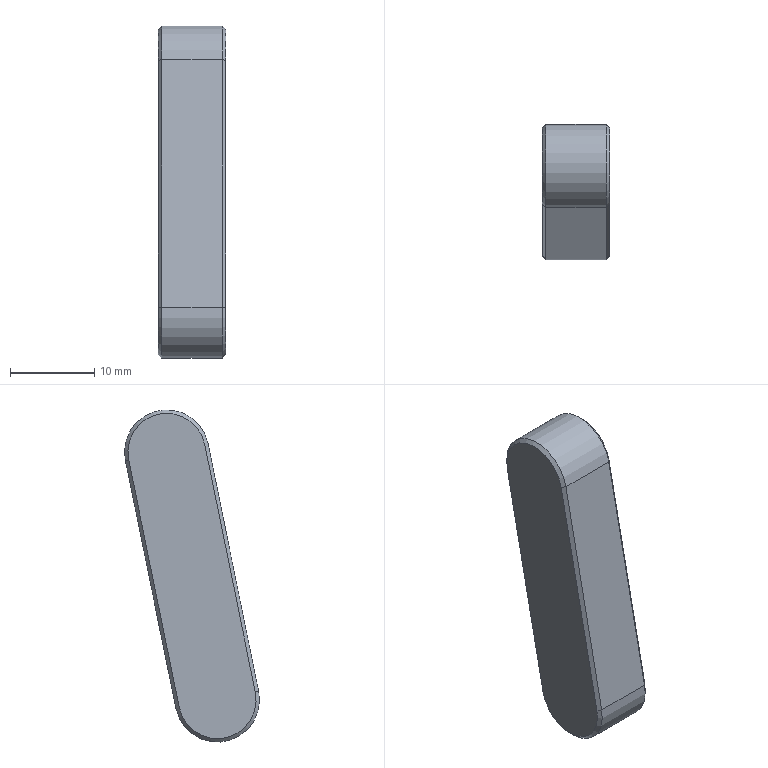Component | SolidWorks | Key_10-40-1 | 1 solid | 14 faces | box 8 x 16 x 39.39 mm | volume 3014 mm3 | plane 8 | cone 4 | cylinder 2 | commonest cylinder face diameters 10 x2
STEP:
#1=COLOUR_RGB('',0.7922,0.8196,0.9333);
#2=FILL_AREA_STYLE_COLOUR('',#1);
#3=FILL_AREA_STYLE('',(#2));
#4=SURFACE_STYLE_FILL_AREA(#3);
#5=SURFACE_SIDE_STYLE('',(#4));
#6=SURFACE_STYLE_USAGE(.BOTH.,#5);
#7=PRESENTATION_STYLE_ASSIGNMENT((#6));
#8=CARTESIAN_POINT('',(0.6063,7.591,5.523));
#9=VERTEX_POINT('',#8);
#10=CARTESIAN_POINT('',(0.8898,7.591,5.523));
#11=VERTEX_POINT('',#10);
#12=CARTESIAN_POINT('',(0.5906,7.591,5.523));
#13=DIRECTION('',(1.,-0.,-0.));
#14=VECTOR('',#13,39.37);
#15=LINE('',#12,#14);
#16=EDGE_CURVE('',#9,#11,#15,.T.);
#17=ORIENTED_EDGE('',*,*,#16,.T.);
#18=CARTESIAN_POINT('',(0.8898,7.828,6.68));
#19=VERTEX_POINT('',#18);
#20=CARTESIAN_POINT('',(0.8898,7.828,6.68));
#21=DIRECTION('',(0.,0.2,0.9798));
#22=VECTOR('',#21,39.37);
#23=LINE('',#20,#22);
#24=EDGE_CURVE('',#11,#19,#23,.T.);
#25=ORIENTED_EDGE('',*,*,#24,.T.);
#26=CARTESIAN_POINT('',(0.6063,7.828,6.68));
#27=VERTEX_POINT('',#26);
#28=CARTESIAN_POINT('',(0.5906,7.828,6.68));
#29=DIRECTION('',(1.,-0.,-0.));
#30=VECTOR('',#29,39.37);
#31=LINE('',#28,#30);
#32=EDGE_CURVE('',#27,#19,#31,.T.);
#33=ORIENTED_EDGE('',*,*,#32,.F.);
#34=CARTESIAN_POINT('',(0.6063,7.552,5.33));
#35=DIRECTION('',(-0.,-0.2,-0.9798));
#36=VECTOR('',#35,39.37);
#37=LINE('',#34,#36);
#38=EDGE_CURVE('',#27,#9,#37,.T.);
#39=ORIENTED_EDGE('',*,*,#38,.T.);
#40=EDGE_LOOP('',(#17,#25,#33,#39));
#41=FACE_OUTER_BOUND('',#40,.T.);
#42=CARTESIAN_POINT('',(0.5906,7.552,5.33));
#43=DIRECTION('',(-0.,0.9798,-0.2));
#44=DIRECTION('',(-0.,-0.2,-0.9798));
#45=AXIS2_PLACEMENT_3D('',#42,#43,#44);
#46=PLANE('',#45);
#47=ADVANCED_FACE('',(#41),#46,.F.);
#48=CARTESIAN_POINT('',(0.6063,8.213,6.601));
#49=VERTEX_POINT('',#48);
#50=CARTESIAN_POINT('',(0.8898,8.213,6.601));
#51=VERTEX_POINT('',#50);
#52=CARTESIAN_POINT('',(0.5906,8.213,6.601));
#53=DIRECTION('',(1.,-0.,-0.));
#54=VECTOR('',#53,39.37);
#55=LINE('',#52,#54);
#56=EDGE_CURVE('',#49,#51,#55,.T.);
#57=ORIENTED_EDGE('',*,*,#56,.T.);
#58=CARTESIAN_POINT('',(0.8898,7.977,5.444));
#59=VERTEX_POINT('',#58);
#60=CARTESIAN_POINT('',(0.8898,7.977,5.444));
#61=DIRECTION('',(-0.,-0.2,-0.9798));
#62=VECTOR('',#61,39.37);
#63=LINE('',#60,#62);
#64=EDGE_CURVE('',#51,#59,#63,.T.);
#65=ORIENTED_EDGE('',*,*,#64,.T.);
#66=CARTESIAN_POINT('',(0.6063,7.977,5.444));
#67=VERTEX_POINT('',#66);
#68=CARTESIAN_POINT('',(0.5906,7.977,5.444));
#69=DIRECTION('',(1.,-0.,-0.));
#70=VECTOR('',#69,39.37);
#71=LINE('',#68,#70);
#72=EDGE_CURVE('',#67,#59,#71,.T.);
#73=ORIENTED_EDGE('',*,*,#72,.F.);
#74=CARTESIAN_POINT('',(0.6063,7.938,5.251));
#75=DIRECTION('',(0.,0.2,0.9798));
#76=VECTOR('',#75,39.37);
#77=LINE('',#74,#76);
#78=EDGE_CURVE('',#67,#49,#77,.T.);
#79=ORIENTED_EDGE('',*,*,#78,.T.);
#80=EDGE_LOOP('',(#57,#65,#73,#79));
#81=FACE_OUTER_BOUND('',#80,.T.);
#82=CARTESIAN_POINT('',(0.5906,7.938,5.251));
#83=DIRECTION('',(0.,-0.9798,0.2));
#84=DIRECTION('',(0.,0.2,0.9798));
#85=AXIS2_PLACEMENT_3D('',#82,#83,#84);
#86=PLANE('',#85);
#87=ADVANCED_FACE('',(#81),#86,.F.);
#88=CARTESIAN_POINT('',(0.5906,7.843,6.677));
#89=VERTEX_POINT('',#88);
#90=CARTESIAN_POINT('',(0.5906,8.198,6.604));
#91=VERTEX_POINT('',#90);
#92=CARTESIAN_POINT('',(0.5906,8.02,6.64));
#93=DIRECTION('',(-1.,0.,0.));
#94=DIRECTION('',(0.,0.9798,-0.2));
#95=AXIS2_PLACEMENT_3D('',#92,#93,#94);
#96=CIRCLE('',#95,0.1811);
#97=EDGE_CURVE('',#89,#91,#96,.T.);
#98=ORIENTED_EDGE('',*,*,#97,.T.);
#99=CARTESIAN_POINT('',(0.5906,7.962,5.447));
#100=VERTEX_POINT('',#99);
#101=CARTESIAN_POINT('',(0.5906,7.922,5.254));
#102=DIRECTION('',(-0.,-0.2,-0.9798));
#103=VECTOR('',#102,39.37);
#104=LINE('',#101,#103);
#105=EDGE_CURVE('',#91,#100,#104,.T.);
#106=ORIENTED_EDGE('',*,*,#105,.T.);
#107=CARTESIAN_POINT('',(0.5906,7.607,5.519));
#108=VERTEX_POINT('',#107);
#109=CARTESIAN_POINT('',(0.5906,7.784,5.483));
#110=DIRECTION('',(-1.,0.,0.));
#111=DIRECTION('',(0.,0.9798,-0.2));
#112=AXIS2_PLACEMENT_3D('',#109,#110,#111);
#113=CIRCLE('',#112,0.1811);
#114=EDGE_CURVE('',#100,#108,#113,.T.);
#115=ORIENTED_EDGE('',*,*,#114,.T.);
#116=CARTESIAN_POINT('',(0.5906,7.568,5.326));
#117=DIRECTION('',(0.,0.2,0.9798));
#118=VECTOR('',#117,39.37);
#119=LINE('',#116,#118);
#120=EDGE_CURVE('',#108,#89,#119,.T.);
#121=ORIENTED_EDGE('',*,*,#120,.T.);
#122=EDGE_LOOP('',(#98,#106,#115,#121));
#123=FACE_OUTER_BOUND('',#122,.T.);
#124=CARTESIAN_POINT('',(0.5906,7.938,5.251));
#125=DIRECTION('',(1.,-0.,-0.));
#126=DIRECTION('',(0.,0.9798,-0.2));
#127=AXIS2_PLACEMENT_3D('',#124,#125,#126);
#128=PLANE('',#127);
#129=ADVANCED_FACE('',(#123),#128,.F.);
#130=CARTESIAN_POINT('',(0.9055,7.843,6.677));
#131=VERTEX_POINT('',#130);
#132=CARTESIAN_POINT('',(0.9055,7.607,5.519));
#133=VERTEX_POINT('',#132);
#134=CARTESIAN_POINT('',(0.9055,7.607,5.519));
#135=DIRECTION('',(-0.,-0.2,-0.9798));
#136=VECTOR('',#135,39.37);
#137=LINE('',#134,#136);
#138=EDGE_CURVE('',#131,#133,#137,.T.);
#139=ORIENTED_EDGE('',*,*,#138,.T.);
#140=CARTESIAN_POINT('',(0.9055,7.962,5.447));
#141=VERTEX_POINT('',#140);
#142=CARTESIAN_POINT('',(0.9055,7.784,5.483));
#143=DIRECTION('',(1.,-0.,-0.));
#144=DIRECTION('',(0.,0.9798,-0.2));
#145=AXIS2_PLACEMENT_3D('',#142,#143,#144);
#146=CIRCLE('',#145,0.1811);
#147=EDGE_CURVE('',#133,#141,#146,.T.);
#148=ORIENTED_EDGE('',*,*,#147,.T.);
#149=CARTESIAN_POINT('',(0.9055,8.198,6.604));
#150=VERTEX_POINT('',#149);
#151=CARTESIAN_POINT('',(0.9055,8.198,6.604));
#152=DIRECTION('',(0.,0.2,0.9798));
#153=VECTOR('',#152,39.37);
#154=LINE('',#151,#153);
#155=EDGE_CURVE('',#141,#150,#154,.T.);
#156=ORIENTED_EDGE('',*,*,#155,.T.);
#157=CARTESIAN_POINT('',(0.9055,8.02,6.64));
#158=DIRECTION('',(1.,-0.,-0.));
#159=DIRECTION('',(0.,0.9798,-0.2));
#160=AXIS2_PLACEMENT_3D('',#157,#158,#159);
#161=CIRCLE('',#160,0.1811);
#162=EDGE_CURVE('',#150,#131,#161,.T.);
#163=ORIENTED_EDGE('',*,*,#162,.T.);
#164=EDGE_LOOP('',(#139,#148,#156,#163));
#165=FACE_OUTER_BOUND('',#164,.T.);
#166=CARTESIAN_POINT('',(0.9055,7.938,5.251));
#167=DIRECTION('',(1.,-0.,-0.));
#168=DIRECTION('',(0.,0.9798,-0.2));
#169=AXIS2_PLACEMENT_3D('',#166,#167,#168);
#170=PLANE('',#169);
#171=ADVANCED_FACE('',(#165),#170,.T.);
#172=ORIENTED_EDGE('',*,*,#32,.T.);
#173=CARTESIAN_POINT('',(0.8898,8.02,6.64));
#174=DIRECTION('',(-1.,0.,0.));
#175=DIRECTION('',(0.,0.9798,-0.2));
#176=AXIS2_PLACEMENT_3D('',#173,#174,#175);
#177=CIRCLE('',#176,0.1969);
#178=EDGE_CURVE('',#19,#51,#177,.T.);
#179=ORIENTED_EDGE('',*,*,#178,.T.);
#180=ORIENTED_EDGE('',*,*,#56,.F.);
#181=CARTESIAN_POINT('',(0.6063,8.02,6.64));
#182=DIRECTION('',(1.,-0.,-0.));
#183=DIRECTION('',(0.,0.9798,-0.2));
#184=AXIS2_PLACEMENT_3D('',#181,#182,#183);
#185=CIRCLE('',#184,0.1969);
#186=EDGE_CURVE('',#49,#27,#185,.T.);
#187=ORIENTED_EDGE('',*,*,#186,.T.);
#188=EDGE_LOOP('',(#172,#179,#180,#187));
#189=FACE_OUTER_BOUND('',#188,.T.);
#190=CARTESIAN_POINT('',(0.5906,8.02,6.64));
#191=DIRECTION('',(1.,-0.,-0.));
#192=DIRECTION('',(0.,0.9798,-0.2));
#193=AXIS2_PLACEMENT_3D('',#190,#191,#192);
#194=CYLINDRICAL_SURFACE('',#193,0.1969);
#195=ADVANCED_FACE('',(#189),#194,.T.);
#196=ORIENTED_EDGE('',*,*,#72,.T.);
#197=CARTESIAN_POINT('',(0.8898,7.784,5.483));
#198=DIRECTION('',(-1.,0.,0.));
#199=DIRECTION('',(0.,0.9798,-0.2));
#200=AXIS2_PLACEMENT_3D('',#197,#198,#199);
#201=CIRCLE('',#200,0.1969);
#202=EDGE_CURVE('',#59,#11,#201,.T.);
#203=ORIENTED_EDGE('',*,*,#202,.T.);
#204=ORIENTED_EDGE('',*,*,#16,.F.);
#205=CARTESIAN_POINT('',(0.6063,7.784,5.483));
#206=DIRECTION('',(1.,-0.,-0.));
#207=DIRECTION('',(0.,0.9798,-0.2));
#208=AXIS2_PLACEMENT_3D('',#205,#206,#207);
#209=CIRCLE('',#208,0.1969);
#210=EDGE_CURVE('',#9,#67,#209,.T.);
#211=ORIENTED_EDGE('',*,*,#210,.T.);
#212=EDGE_LOOP('',(#196,#203,#204,#211));
#213=FACE_OUTER_BOUND('',#212,.T.);
#214=CARTESIAN_POINT('',(0.5906,7.784,5.483));
#215=DIRECTION('',(1.,-0.,-0.));
#216=DIRECTION('',(0.,0.9798,-0.2));
#217=AXIS2_PLACEMENT_3D('',#214,#215,#216);
#218=CYLINDRICAL_SURFACE('',#217,0.1969);
#219=ADVANCED_FACE('',(#213),#218,.T.);
#220=CARTESIAN_POINT('',(0.9055,7.843,6.677));
#221=DIRECTION('',(-0.7071,-0.6928,0.1414));
#222=VECTOR('',#221,39.37);
#223=LINE('',#220,#222);
#224=EDGE_CURVE('',#131,#19,#223,.T.);
#225=ORIENTED_EDGE('',*,*,#224,.F.);
#226=ORIENTED_EDGE('',*,*,#162,.F.);
#227=CARTESIAN_POINT('',(0.8898,8.213,6.601));
#228=DIRECTION('',(0.7071,-0.6928,0.1414));
#229=VECTOR('',#228,39.37);
#230=LINE('',#227,#229);
#231=EDGE_CURVE('',#51,#150,#230,.T.);
#232=ORIENTED_EDGE('',*,*,#231,.F.);
#233=ORIENTED_EDGE('',*,*,#178,.F.);
#234=EDGE_LOOP('',(#225,#226,#232,#233));
#235=FACE_OUTER_BOUND('',#234,.T.);
#236=CARTESIAN_POINT('',(0.8898,8.02,6.64));
#237=DIRECTION('',(-1.,0.,0.));
#238=DIRECTION('',(0.,-0.9798,0.2));
#239=AXIS2_PLACEMENT_3D('',#236,#237,#238);
#240=CONICAL_SURFACE('',#239,0.1969,0.7854);
#241=ADVANCED_FACE('',(#235),#240,.T.);
#242=ORIENTED_EDGE('',*,*,#231,.T.);
#243=ORIENTED_EDGE('',*,*,#155,.F.);
#244=CARTESIAN_POINT('',(0.8898,7.977,5.444));
#245=DIRECTION('',(0.7071,-0.6928,0.1414));
#246=VECTOR('',#245,39.37);
#247=LINE('',#244,#246);
#248=EDGE_CURVE('',#59,#141,#247,.T.);
#249=ORIENTED_EDGE('',*,*,#248,.F.);
#250=ORIENTED_EDGE('',*,*,#64,.F.);
#251=EDGE_LOOP('',(#242,#243,#249,#250));
#252=FACE_OUTER_BOUND('',#251,.T.);
#253=CARTESIAN_POINT('',(0.8898,7.938,5.251));
#254=DIRECTION('',(0.7071,0.6928,-0.1414));
#255=DIRECTION('',(-0.7071,0.6928,-0.1414));
#256=AXIS2_PLACEMENT_3D('',#253,#254,#255);
#257=PLANE('',#256);
#258=ADVANCED_FACE('',(#252),#257,.T.);
#259=ORIENTED_EDGE('',*,*,#224,.T.);
#260=ORIENTED_EDGE('',*,*,#24,.F.);
#261=CARTESIAN_POINT('',(0.9055,7.607,5.519));
#262=DIRECTION('',(-0.7071,-0.6928,0.1414));
#263=VECTOR('',#262,39.37);
#264=LINE('',#261,#263);
#265=EDGE_CURVE('',#133,#11,#264,.T.);
#266=ORIENTED_EDGE('',*,*,#265,.F.);
#267=ORIENTED_EDGE('',*,*,#138,.F.);
#268=EDGE_LOOP('',(#259,#260,#266,#267));
#269=FACE_OUTER_BOUND('',#268,.T.);
#270=CARTESIAN_POINT('',(0.8898,7.552,5.33));
#271=DIRECTION('',(0.7071,-0.6928,0.1414));
#272=DIRECTION('',(0.7071,0.6928,-0.1414));
#273=AXIS2_PLACEMENT_3D('',#270,#271,#272);
#274=PLANE('',#273);
#275=ADVANCED_FACE('',(#269),#274,.T.);
#276=ORIENTED_EDGE('',*,*,#248,.T.);
#277=ORIENTED_EDGE('',*,*,#147,.F.);
#278=ORIENTED_EDGE('',*,*,#265,.T.);
#279=ORIENTED_EDGE('',*,*,#202,.F.);
#280=EDGE_LOOP('',(#276,#277,#278,#279));
#281=FACE_OUTER_BOUND('',#280,.T.);
#282=CARTESIAN_POINT('',(0.8898,7.784,5.483));
#283=DIRECTION('',(-1.,0.,0.));
#284=DIRECTION('',(0.,-0.9798,0.2));
#285=AXIS2_PLACEMENT_3D('',#282,#283,#284);
#286=CONICAL_SURFACE('',#285,0.1969,0.7854);
#287=ADVANCED_FACE('',(#281),#286,.T.);
#288=CARTESIAN_POINT('',(0.6063,7.591,5.523));
#289=DIRECTION('',(-0.7071,0.6928,-0.1414));
#290=VECTOR('',#289,39.37);
#291=LINE('',#288,#290);
#292=EDGE_CURVE('',#9,#108,#291,.T.);
#293=ORIENTED_EDGE('',*,*,#292,.F.);
#294=ORIENTED_EDGE('',*,*,#38,.F.);
#295=CARTESIAN_POINT('',(0.5906,7.843,6.677));
#296=DIRECTION('',(0.7071,-0.6928,0.1414));
#297=VECTOR('',#296,39.37);
#298=LINE('',#295,#297);
#299=EDGE_CURVE('',#89,#27,#298,.T.);
#300=ORIENTED_EDGE('',*,*,#299,.F.);
#301=ORIENTED_EDGE('',*,*,#120,.F.);
#302=EDGE_LOOP('',(#293,#294,#300,#301));
#303=FACE_OUTER_BOUND('',#302,.T.);
#304=CARTESIAN_POINT('',(0.5906,7.568,5.326));
#305=DIRECTION('',(0.7071,0.6928,-0.1414));
#306=DIRECTION('',(-0.7071,0.6928,-0.1414));
#307=AXIS2_PLACEMENT_3D('',#304,#305,#306);
#308=PLANE('',#307);
#309=ADVANCED_FACE('',(#303),#308,.F.);
#310=ORIENTED_EDGE('',*,*,#299,.T.);
#311=ORIENTED_EDGE('',*,*,#186,.F.);
#312=CARTESIAN_POINT('',(0.5906,8.198,6.604));
#313=DIRECTION('',(0.7071,0.6928,-0.1414));
#314=VECTOR('',#313,39.37);
#315=LINE('',#312,#314);
#316=EDGE_CURVE('',#91,#49,#315,.T.);
#317=ORIENTED_EDGE('',*,*,#316,.F.);
#318=ORIENTED_EDGE('',*,*,#97,.F.);
#319=EDGE_LOOP('',(#310,#311,#317,#318));
#320=FACE_OUTER_BOUND('',#319,.T.);
#321=CARTESIAN_POINT('',(0.5906,8.02,6.64));
#322=DIRECTION('',(1.,-0.,-0.));
#323=DIRECTION('',(0.,0.9798,-0.2));
#324=AXIS2_PLACEMENT_3D('',#321,#322,#323);
#325=CONICAL_SURFACE('',#324,0.1811,0.7854);
#326=ADVANCED_FACE('',(#320),#325,.T.);
#327=ORIENTED_EDGE('',*,*,#292,.T.);
#328=ORIENTED_EDGE('',*,*,#114,.F.);
#329=CARTESIAN_POINT('',(0.6063,7.977,5.444));
#330=DIRECTION('',(-0.7071,-0.6928,0.1414));
#331=VECTOR('',#330,39.37);
#332=LINE('',#329,#331);
#333=EDGE_CURVE('',#67,#100,#332,.T.);
#334=ORIENTED_EDGE('',*,*,#333,.F.);
#335=ORIENTED_EDGE('',*,*,#210,.F.);
#336=EDGE_LOOP('',(#327,#328,#334,#335));
#337=FACE_OUTER_BOUND('',#336,.T.);
#338=CARTESIAN_POINT('',(0.5906,7.784,5.483));
#339=DIRECTION('',(1.,-0.,-0.));
#340=DIRECTION('',(0.,0.9798,-0.2));
#341=AXIS2_PLACEMENT_3D('',#338,#339,#340);
#342=CONICAL_SURFACE('',#341,0.1811,0.7854);
#343=ADVANCED_FACE('',(#337),#342,.T.);
#344=ORIENTED_EDGE('',*,*,#316,.T.);
#345=ORIENTED_EDGE('',*,*,#78,.F.);
#346=ORIENTED_EDGE('',*,*,#333,.T.);
#347=ORIENTED_EDGE('',*,*,#105,.F.);
#348=EDGE_LOOP('',(#344,#345,#346,#347));
#349=FACE_OUTER_BOUND('',#348,.T.);
#350=CARTESIAN_POINT('',(0.5906,7.922,5.254));
#351=DIRECTION('',(0.7071,-0.6928,0.1414));
#352=DIRECTION('',(0.7071,0.6928,-0.1414));
#353=AXIS2_PLACEMENT_3D('',#350,#351,#352);
#354=PLANE('',#353);
#355=ADVANCED_FACE('',(#349),#354,.F.);
#356=CLOSED_SHELL('',(#47,#87,#129,#171,#195,#219,#241,#258,#275,#287,#309,#326,#343,#355));
#357=MANIFOLD_SOLID_BREP('',#356);
#358=STYLED_ITEM('',(#7),#357);
#359=PRESENTATION_LAYER_ASSIGNMENT('','',(#358));
#360=CARTESIAN_POINT('',(0.,0.,0.));
#361=DIRECTION('',(0.,0.,1.));
#362=DIRECTION('',(1.,0.,0.));
#363=AXIS2_PLACEMENT_3D('',#360,#361,#362);
#364=(LENGTH_UNIT()NAMED_UNIT(*)SI_UNIT($,.METRE.));
#365=LENGTH_MEASURE_WITH_UNIT(LENGTH_MEASURE(0.0254),#364);
#366=DIMENSIONAL_EXPONENTS(1.,0.,0.,0.,0.,0.,0.);
#367=(CONVERSION_BASED_UNIT('',#365)LENGTH_UNIT()NAMED_UNIT(#366));
#368=UNCERTAINTY_MEASURE_WITH_UNIT(LENGTH_MEASURE(0.00001),#367,'','');
#369=(NAMED_UNIT(*)PLANE_ANGLE_UNIT()SI_UNIT($,.RADIAN.));
#370=(NAMED_UNIT(*)SI_UNIT($,.STERADIAN.)SOLID_ANGLE_UNIT());
#371=(GEOMETRIC_REPRESENTATION_CONTEXT(3)GLOBAL_UNCERTAINTY_ASSIGNED_CONTEXT((#368))GLOBAL_UNIT_ASSIGNED_CONTEXT((#367,#369,#370))REPRESENTATION_CONTEXT('',''));
#372=ADVANCED_BREP_SHAPE_REPRESENTATION('',(#357,#363),#371);
#373=(LENGTH_UNIT()NAMED_UNIT(*)SI_UNIT($,.METRE.));
#374=LENGTH_MEASURE_WITH_UNIT(LENGTH_MEASURE(0.0254),#373);
#375=DIMENSIONAL_EXPONENTS(1.,0.,0.,0.,0.,0.,0.);
#376=(CONVERSION_BASED_UNIT('',#374)LENGTH_UNIT()NAMED_UNIT(#375));
#377=UNCERTAINTY_MEASURE_WITH_UNIT(LENGTH_MEASURE(0.00001),#376,'','');
#378=(NAMED_UNIT(*)PLANE_ANGLE_UNIT()SI_UNIT($,.RADIAN.));
#379=(NAMED_UNIT(*)SI_UNIT($,.STERADIAN.)SOLID_ANGLE_UNIT());
#380=(GEOMETRIC_REPRESENTATION_CONTEXT(3)GLOBAL_UNCERTAINTY_ASSIGNED_CONTEXT((#377))GLOBAL_UNIT_ASSIGNED_CONTEXT((#376,#378,#379))REPRESENTATION_CONTEXT('',''));
#381=MECHANICAL_DESIGN_GEOMETRIC_PRESENTATION_REPRESENTATION('',(#358),#380);